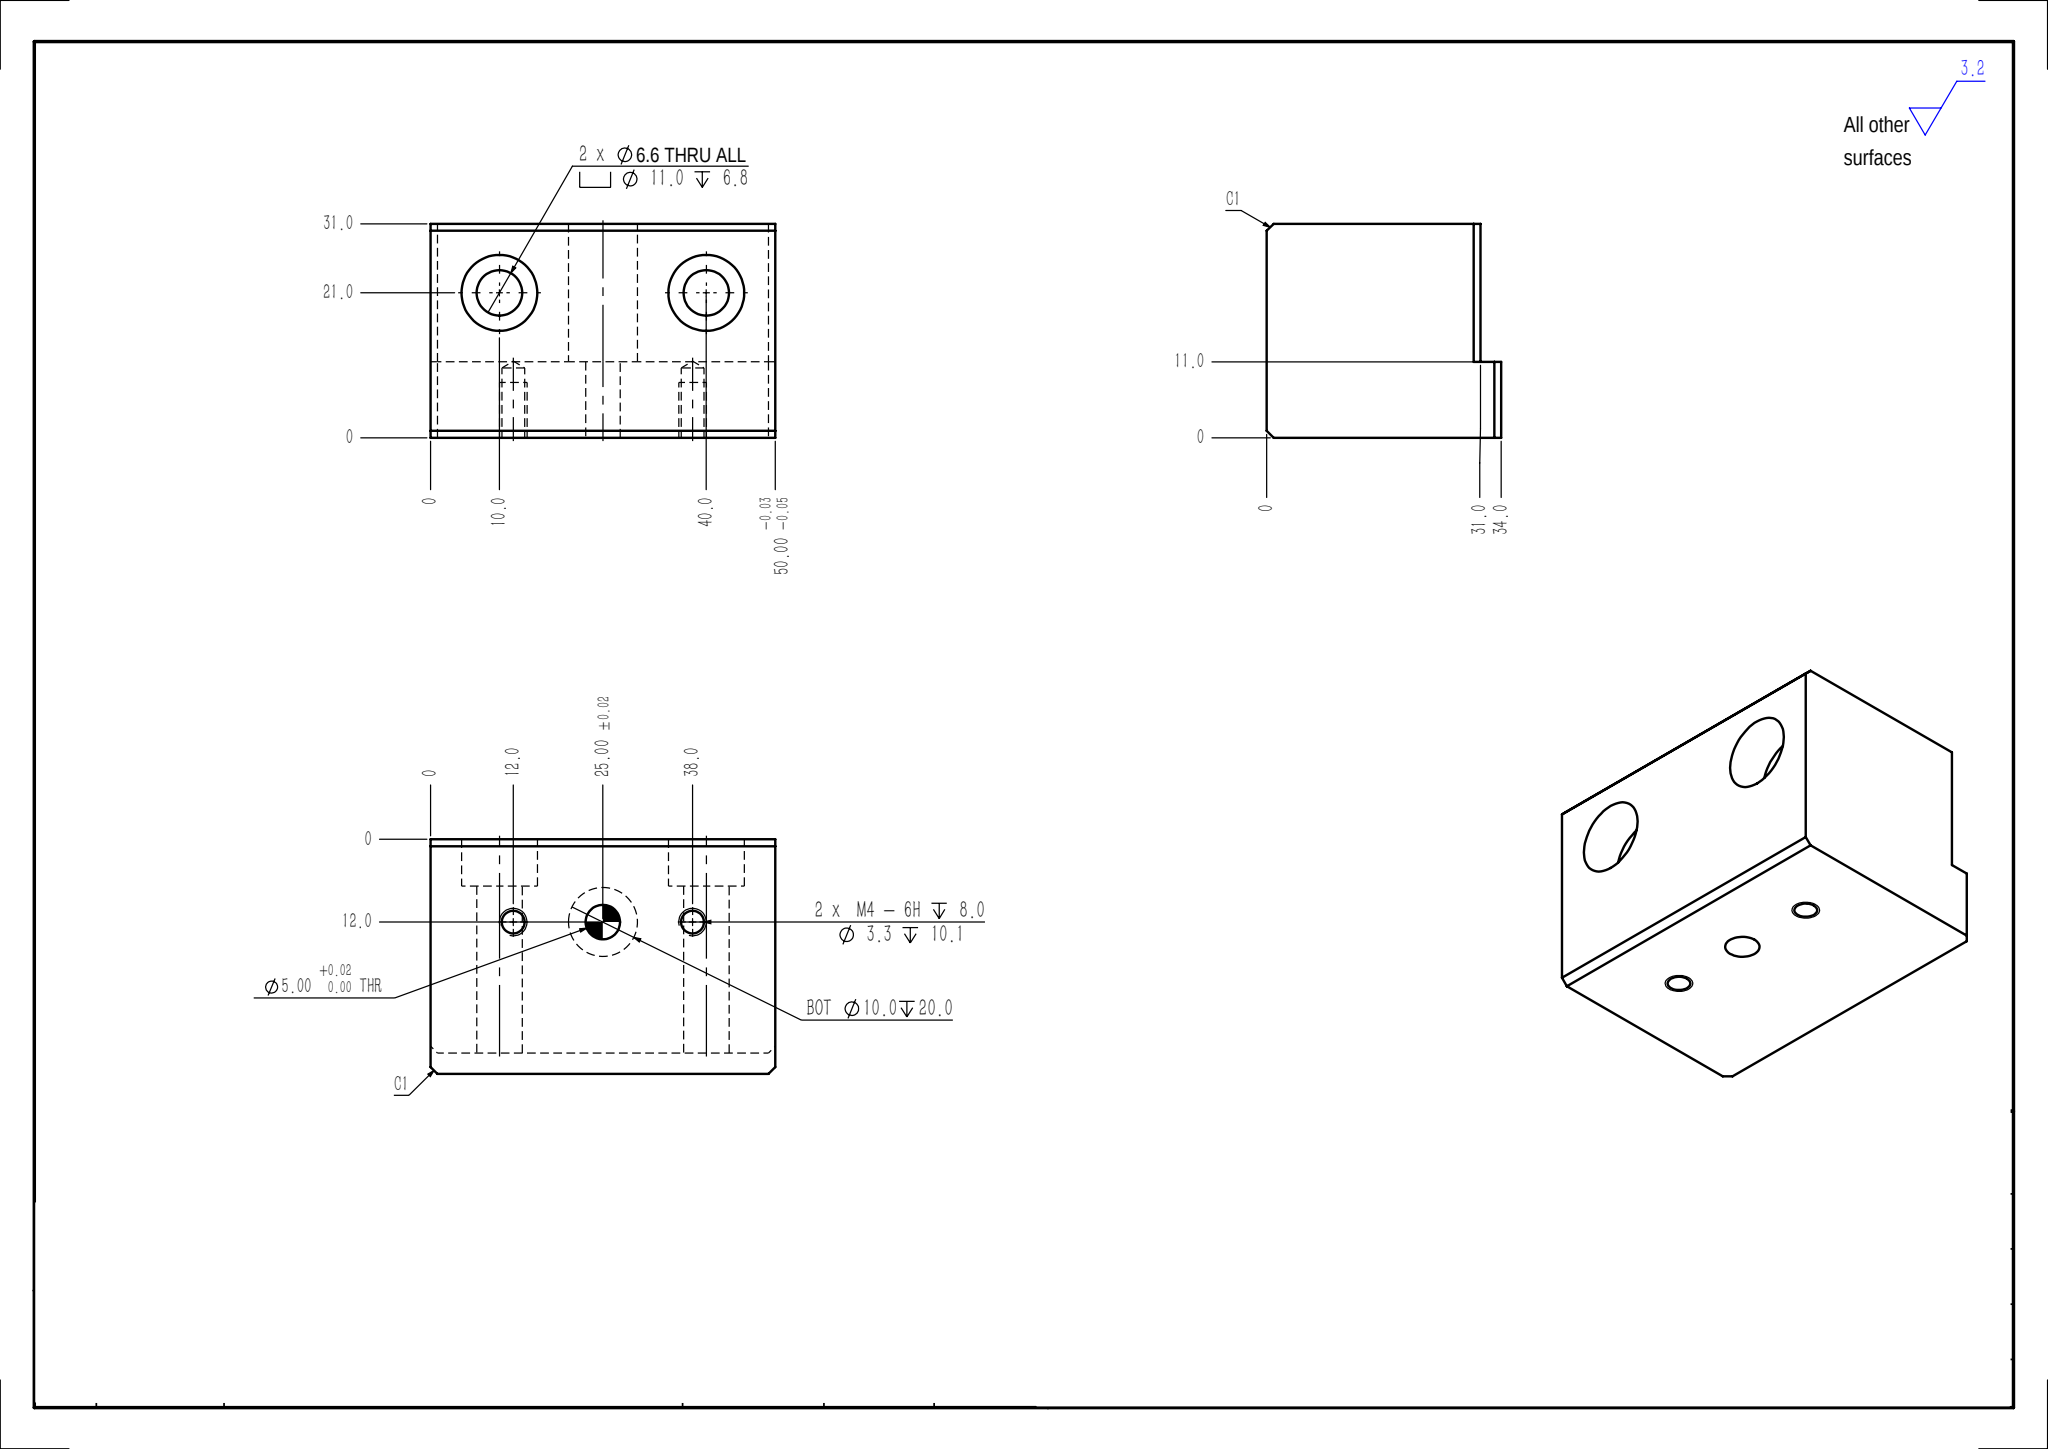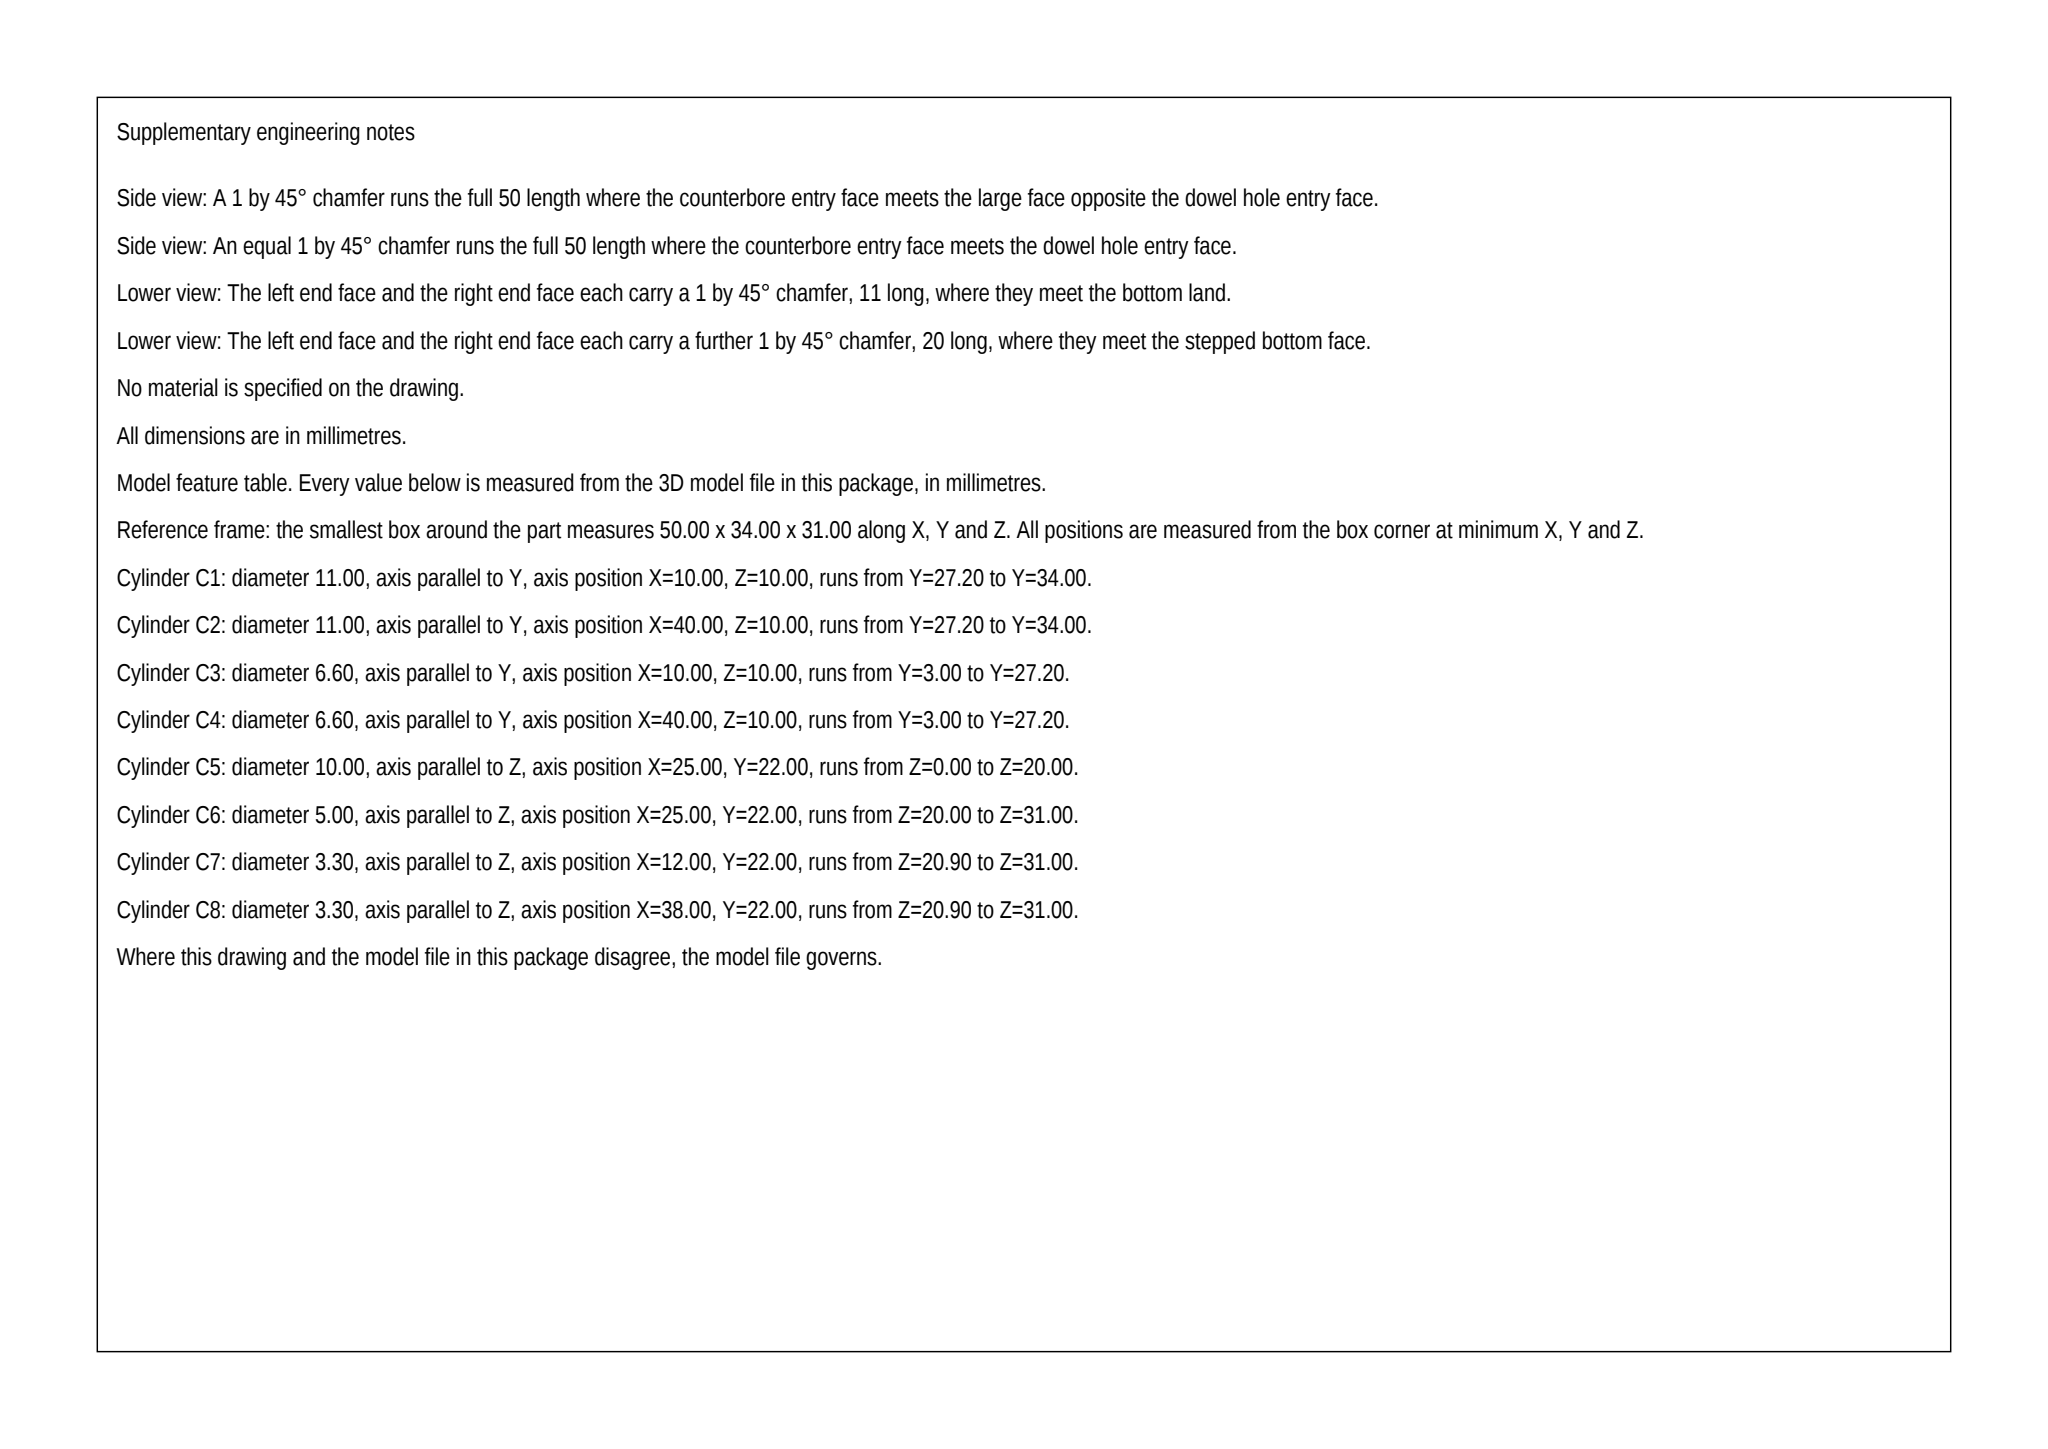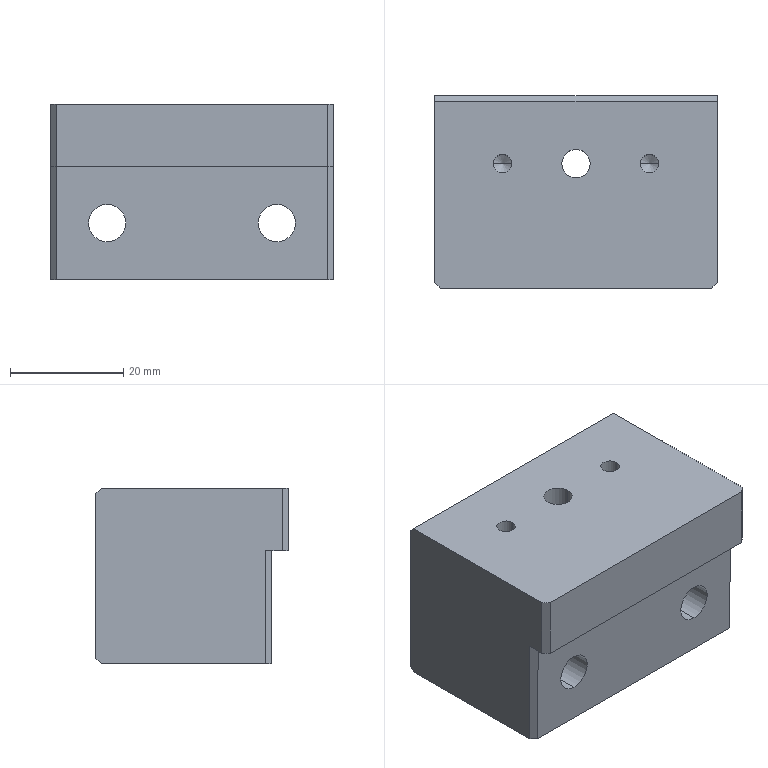Part | SolidWorks | mm | 1 solid | 37 faces | box 50 x 34 x 31 mm | volume 44705 mm3 | plane 17 | cylinder 16 | cone 4 | commonest cylinder face diameters 3.3 x4 11 x4 6.6 x4 10 x2 5 x2
build123d program:
from build123d import *

# Parameters (mm, degrees)
SKETCH1_W                                            = 50
SKETCH1_H                                            = 50
BOSS_EXTRUDE1_DEPTH                                  = 34
SKETCH2_W                                            = 20
SKETCH2_H                                            = 3
CUT_EXTRUDE1_DEPTH                                   = 66.429
SKETCH3_W                                            = 50
SKETCH3_H                                            = 15
CUT_EXTRUDE2_DEPTH                                   = 2
HOLE_SIZE_ACCORDING_TO_TYPE_1_OF_HEXAGON_D           = 6.6
HOLE_SIZE_ACCORDING_TO_TYPE_1_OF_HEXAGON_CBORE_D     = 11
HOLE_SIZE_ACCORDING_TO_TYPE_1_OF_HEXAGON_CBORE_DEPTH = 6.8
SKETCH6_W                                            = 19
SKETCH6_H                                            = 25
CUT_EXTRUDE3_DEPTH                                   = 66.429
SIZE_MM_DOWEL_HOLE1_D                                = 5
M4_TAPPED_HOLE1_D                                    = 3.3
M4_TAPPED_HOLE1_DEPTH                                = 10.1
M4_TAPPED_HOLE1_TIP                                  = 0.9914
SKETCH11_R                                           = 5
CUT_EXTRUDE4_DEPTH                                   = 20
SKETCH12_W                                           = 50
SKETCH12_H                                           = 19
CUT_EXTRUDE5_DEPTH                                   = 44.301
CHAMFER1_SIZE                                        = 1


with BuildPart() as part:
    # Sketch1 → Boss-Extrude1 (new body)
    with BuildSketch(Plane(origin=(0, 0, 0), x_dir=(1, 0, 0), z_dir=(0, 1, 0))):
        Rectangle(SKETCH1_W, SKETCH1_H)
    extrude(amount=BOSS_EXTRUDE1_DEPTH)

    # Sketch2 → Cut-Extrude1 (cut, through all)
    with BuildSketch(Plane(origin=(25, 0, 0), x_dir=(0, 0, -1), z_dir=(1, 0, 0))):
        with Locations((15, 1.5)):
            Rectangle(SKETCH2_W, SKETCH2_H)
    extrude(amount=-CUT_EXTRUDE1_DEPTH, mode=Mode.SUBTRACT)

    # Sketch3 → Cut-Extrude2 (cut)
    with BuildSketch(Plane(origin=(0, 34, 0), x_dir=(1, 0, 0), z_dir=(0, 1, 0))):
        with Locations((0, -15.5)):
            Rectangle(SKETCH3_W, SKETCH3_H)
    extrude(amount=-CUT_EXTRUDE2_DEPTH, mode=Mode.SUBTRACT)

    # Hole Size_According to_Type 1 of Hexagon (through all)
    with Locations(Plane(origin=(0, 34, 0), x_dir=(1, 0, 0), z_dir=(0, 1, 0))):
        with Locations((-15, 15), (15, 15)):
            CounterBoreHole(HOLE_SIZE_ACCORDING_TO_TYPE_1_OF_HEXAGON_D / 2, HOLE_SIZE_ACCORDING_TO_TYPE_1_OF_HEXAGON_CBORE_D / 2, HOLE_SIZE_ACCORDING_TO_TYPE_1_OF_HEXAGON_CBORE_DEPTH)

    # Sketch6 → Cut-Extrude3 (cut, through all)
    with BuildSketch(Plane.ZY.offset(25)):
        with Locations((15.5, 21.5)):
            Rectangle(SKETCH6_W, SKETCH6_H)
    extrude(amount=-CUT_EXTRUDE3_DEPTH, mode=Mode.SUBTRACT)

    # Size mm Dowel Hole1 (through all)
    with Locations(Plane.XY.offset(6)):
        with Locations((0, 22)):
            Hole(SIZE_MM_DOWEL_HOLE1_D / 2)

    # M4 Tapped Hole1
    with Locations(Plane.XY.offset(6)):
        with Locations((-13, 22), (13, 22)):
            Hole(M4_TAPPED_HOLE1_D / 2, depth=M4_TAPPED_HOLE1_DEPTH)
            with Locations((0, 0, -(M4_TAPPED_HOLE1_DEPTH + M4_TAPPED_HOLE1_TIP / 2))):  # 118° drill point
                Cone(0, M4_TAPPED_HOLE1_D / 2, M4_TAPPED_HOLE1_TIP, mode=Mode.SUBTRACT)

    # Sketch11 → Cut-Extrude4 (cut)
    with BuildSketch(Plane(origin=(0, 0, -25), x_dir=(-1, 0, 0), z_dir=(0, 0, -1))):
        with Locations((0, 22)):
            Circle(SKETCH11_R)
    extrude(amount=-CUT_EXTRUDE4_DEPTH, mode=Mode.SUBTRACT)

    # Sketch12 → Cut-Extrude5 (cut, through all)
    with BuildSketch(Plane(origin=(0, 9, 0), x_dir=(1, 0, 0), z_dir=(0, 1, 0))):
        with Locations((0, -15.5)):
            Rectangle(SKETCH12_W, SKETCH12_H)
    extrude(amount=-CUT_EXTRUDE5_DEPTH, mode=Mode.SUBTRACT)

    # Chamfer1
    chamfer1_edges = [part.edges().sort_by_distance(p)[0] for p in [
        (25, 0, 0.5),
        (-25, 0, 0.5),
        (-25, 3, -15),
        (25, 3, -15),
        (0, 34, -25),
        (0, 34, 6),
    ]]
    chamfer(chamfer1_edges, length=CHAMFER1_SIZE)


solid = part.part